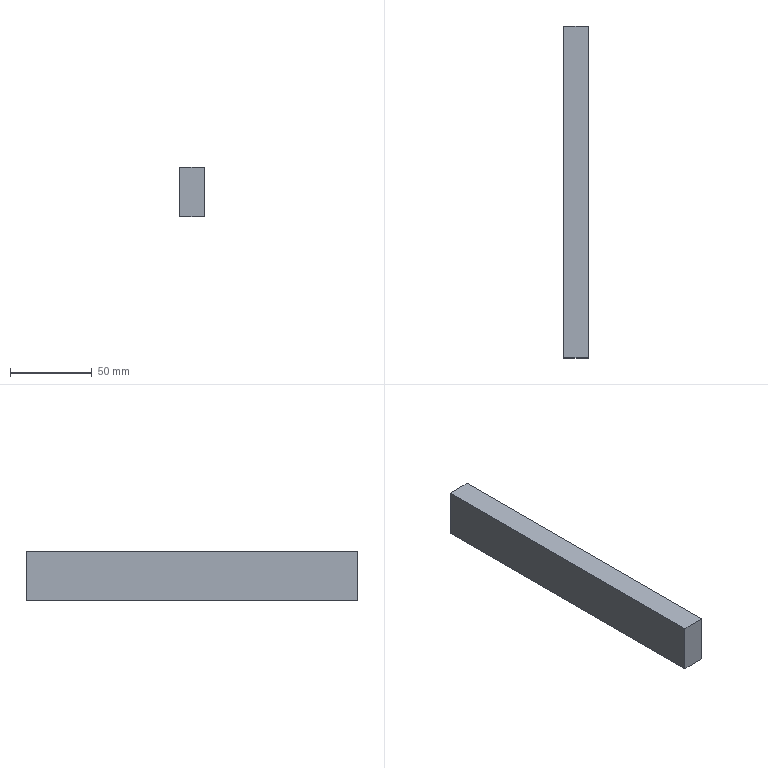Component | SolidWorks | SlideRailFixingPlate-1 | 1 solid | 6 faces | box 14.7 x 203 x 30 mm | volume 89523 mm3 | plane 6
build123d program:
from build123d import *

# Parameters (mm, degrees)
BOSS_EXTRUDE1_DEPTH      = 78
BOSS_EXTRUDE1_DEPTH_BACK = 125
SKETCH2_W                = 30
SKETCH2_H                = 14.7


with BuildPart() as part:
    # Sketch2 → Boss-Extrude1 (new, two sides: drawn at the far end of the back side and taken through both)
    with BuildSketch(Plane.XY.offset(-BOSS_EXTRUDE1_DEPTH_BACK)):
        with Locations((0, 243.349)):
            Rectangle(SKETCH2_W, SKETCH2_H)
    extrude(amount=BOSS_EXTRUDE1_DEPTH + BOSS_EXTRUDE1_DEPTH_BACK)


solid = part.part

# Placed as in the assembly
solid = solid.moved(Location((-235.297, 103.983, 271.626), (90, 0, 90)))
STEP:
#1=COLOUR_RGB('',0.7922,0.8196,0.9333);
#2=FILL_AREA_STYLE_COLOUR('',#1);
#3=FILL_AREA_STYLE('',(#2));
#4=SURFACE_STYLE_FILL_AREA(#3);
#5=SURFACE_SIDE_STYLE('',(#4));
#6=SURFACE_STYLE_USAGE(.BOTH.,#5);
#7=PRESENTATION_STYLE_ASSIGNMENT((#6));
#8=CARTESIAN_POINT('',(-19.134,1.023,11.284));
#9=VERTEX_POINT('',#8);
#10=CARTESIAN_POINT('',(-19.134,9.015,11.284));
#11=VERTEX_POINT('',#10);
#12=CARTESIAN_POINT('',(-19.134,1.023,11.284));
#13=DIRECTION('',(-0.,1.,-0.));
#14=VECTOR('',#13,39.37);
#15=LINE('',#12,#14);
#16=EDGE_CURVE('',#9,#11,#15,.T.);
#17=ORIENTED_EDGE('',*,*,#16,.T.);
#18=CARTESIAN_POINT('',(-19.134,9.015,10.103));
#19=VERTEX_POINT('',#18);
#20=CARTESIAN_POINT('',(-19.134,9.015,10.103));
#21=DIRECTION('',(-0.,0.,1.));
#22=VECTOR('',#21,39.37);
#23=LINE('',#20,#22);
#24=EDGE_CURVE('',#19,#11,#23,.T.);
#25=ORIENTED_EDGE('',*,*,#24,.F.);
#26=CARTESIAN_POINT('',(-19.134,1.023,10.103));
#27=VERTEX_POINT('',#26);
#28=CARTESIAN_POINT('',(-19.134,1.023,10.103));
#29=DIRECTION('',(-0.,1.,-0.));
#30=VECTOR('',#29,39.37);
#31=LINE('',#28,#30);
#32=EDGE_CURVE('',#27,#19,#31,.T.);
#33=ORIENTED_EDGE('',*,*,#32,.F.);
#34=CARTESIAN_POINT('',(-19.134,1.023,10.103));
#35=DIRECTION('',(-0.,0.,1.));
#36=VECTOR('',#35,39.37);
#37=LINE('',#34,#36);
#38=EDGE_CURVE('',#27,#9,#37,.T.);
#39=ORIENTED_EDGE('',*,*,#38,.T.);
#40=EDGE_LOOP('',(#17,#25,#33,#39));
#41=FACE_OUTER_BOUND('',#40,.T.);
#42=CARTESIAN_POINT('',(-19.134,1.023,10.103));
#43=DIRECTION('',(-1.,-0.,-0.));
#44=DIRECTION('',(-0.,1.,-0.));
#45=AXIS2_PLACEMENT_3D('',#42,#43,#44);
#46=PLANE('',#45);
#47=ADVANCED_FACE('',(#41),#46,.T.);
#48=ORIENTED_EDGE('',*,*,#32,.T.);
#49=CARTESIAN_POINT('',(-18.555,9.015,10.103));
#50=VERTEX_POINT('',#49);
#51=CARTESIAN_POINT('',(-18.555,9.015,10.103));
#52=DIRECTION('',(-1.,-0.,-0.));
#53=VECTOR('',#52,39.37);
#54=LINE('',#51,#53);
#55=EDGE_CURVE('',#50,#19,#54,.T.);
#56=ORIENTED_EDGE('',*,*,#55,.F.);
#57=CARTESIAN_POINT('',(-18.555,1.023,10.103));
#58=VERTEX_POINT('',#57);
#59=CARTESIAN_POINT('',(-18.555,1.023,10.103));
#60=DIRECTION('',(-0.,1.,-0.));
#61=VECTOR('',#60,39.37);
#62=LINE('',#59,#61);
#63=EDGE_CURVE('',#58,#50,#62,.T.);
#64=ORIENTED_EDGE('',*,*,#63,.F.);
#65=CARTESIAN_POINT('',(-18.555,1.023,10.103));
#66=DIRECTION('',(-1.,-0.,-0.));
#67=VECTOR('',#66,39.37);
#68=LINE('',#65,#67);
#69=EDGE_CURVE('',#58,#27,#68,.T.);
#70=ORIENTED_EDGE('',*,*,#69,.T.);
#71=EDGE_LOOP('',(#48,#56,#64,#70));
#72=FACE_OUTER_BOUND('',#71,.T.);
#73=CARTESIAN_POINT('',(-18.555,1.023,10.103));
#74=DIRECTION('',(0.,-0.,-1.));
#75=DIRECTION('',(0.,-1.,0.));
#76=AXIS2_PLACEMENT_3D('',#73,#74,#75);
#77=PLANE('',#76);
#78=ADVANCED_FACE('',(#72),#77,.T.);
#79=ORIENTED_EDGE('',*,*,#63,.T.);
#80=CARTESIAN_POINT('',(-18.555,9.015,11.284));
#81=VERTEX_POINT('',#80);
#82=CARTESIAN_POINT('',(-18.555,9.015,10.103));
#83=DIRECTION('',(-0.,0.,1.));
#84=VECTOR('',#83,39.37);
#85=LINE('',#82,#84);
#86=EDGE_CURVE('',#50,#81,#85,.T.);
#87=ORIENTED_EDGE('',*,*,#86,.T.);
#88=CARTESIAN_POINT('',(-18.555,1.023,11.284));
#89=VERTEX_POINT('',#88);
#90=CARTESIAN_POINT('',(-18.555,1.023,11.284));
#91=DIRECTION('',(-0.,1.,-0.));
#92=VECTOR('',#91,39.37);
#93=LINE('',#90,#92);
#94=EDGE_CURVE('',#89,#81,#93,.T.);
#95=ORIENTED_EDGE('',*,*,#94,.F.);
#96=CARTESIAN_POINT('',(-18.555,1.023,10.103));
#97=DIRECTION('',(-0.,0.,1.));
#98=VECTOR('',#97,39.37);
#99=LINE('',#96,#98);
#100=EDGE_CURVE('',#58,#89,#99,.T.);
#101=ORIENTED_EDGE('',*,*,#100,.F.);
#102=EDGE_LOOP('',(#79,#87,#95,#101));
#103=FACE_OUTER_BOUND('',#102,.T.);
#104=CARTESIAN_POINT('',(-18.555,1.023,10.103));
#105=DIRECTION('',(-1.,-0.,-0.));
#106=DIRECTION('',(-0.,1.,-0.));
#107=AXIS2_PLACEMENT_3D('',#104,#105,#106);
#108=PLANE('',#107);
#109=ADVANCED_FACE('',(#103),#108,.F.);
#110=ORIENTED_EDGE('',*,*,#94,.T.);
#111=CARTESIAN_POINT('',(-18.555,9.015,11.284));
#112=DIRECTION('',(-1.,-0.,-0.));
#113=VECTOR('',#112,39.37);
#114=LINE('',#111,#113);
#115=EDGE_CURVE('',#81,#11,#114,.T.);
#116=ORIENTED_EDGE('',*,*,#115,.T.);
#117=ORIENTED_EDGE('',*,*,#16,.F.);
#118=CARTESIAN_POINT('',(-18.555,1.023,11.284));
#119=DIRECTION('',(-1.,-0.,-0.));
#120=VECTOR('',#119,39.37);
#121=LINE('',#118,#120);
#122=EDGE_CURVE('',#89,#9,#121,.T.);
#123=ORIENTED_EDGE('',*,*,#122,.F.);
#124=EDGE_LOOP('',(#110,#116,#117,#123));
#125=FACE_OUTER_BOUND('',#124,.T.);
#126=CARTESIAN_POINT('',(-18.555,1.023,11.284));
#127=DIRECTION('',(0.,-0.,-1.));
#128=DIRECTION('',(0.,-1.,0.));
#129=AXIS2_PLACEMENT_3D('',#126,#127,#128);
#130=PLANE('',#129);
#131=ADVANCED_FACE('',(#125),#130,.F.);
#132=ORIENTED_EDGE('',*,*,#38,.F.);
#133=ORIENTED_EDGE('',*,*,#69,.F.);
#134=ORIENTED_EDGE('',*,*,#100,.T.);
#135=ORIENTED_EDGE('',*,*,#122,.T.);
#136=EDGE_LOOP('',(#132,#133,#134,#135));
#137=FACE_OUTER_BOUND('',#136,.T.);
#138=CARTESIAN_POINT('',(-9.264,1.023,10.694));
#139=DIRECTION('',(0.,-1.,0.));
#140=DIRECTION('',(-0.,0.,1.));
#141=AXIS2_PLACEMENT_3D('',#138,#139,#140);
#142=PLANE('',#141);
#143=ADVANCED_FACE('',(#137),#142,.T.);
#144=ORIENTED_EDGE('',*,*,#24,.T.);
#145=ORIENTED_EDGE('',*,*,#115,.F.);
#146=ORIENTED_EDGE('',*,*,#86,.F.);
#147=ORIENTED_EDGE('',*,*,#55,.T.);
#148=EDGE_LOOP('',(#144,#145,#146,#147));
#149=FACE_OUTER_BOUND('',#148,.T.);
#150=CARTESIAN_POINT('',(-9.264,9.015,10.694));
#151=DIRECTION('',(0.,-1.,0.));
#152=DIRECTION('',(-0.,0.,1.));
#153=AXIS2_PLACEMENT_3D('',#150,#151,#152);
#154=PLANE('',#153);
#155=ADVANCED_FACE('',(#149),#154,.F.);
#156=CLOSED_SHELL('',(#47,#78,#109,#131,#143,#155));
#157=MANIFOLD_SOLID_BREP('',#156);
#158=STYLED_ITEM('',(#7),#157);
#159=PRESENTATION_LAYER_ASSIGNMENT('','',(#158));
#160=CARTESIAN_POINT('',(0.,0.,0.));
#161=DIRECTION('',(0.,0.,1.));
#162=DIRECTION('',(1.,0.,0.));
#163=AXIS2_PLACEMENT_3D('',#160,#161,#162);
#164=(LENGTH_UNIT()NAMED_UNIT(*)SI_UNIT($,.METRE.));
#165=LENGTH_MEASURE_WITH_UNIT(LENGTH_MEASURE(0.0254),#164);
#166=DIMENSIONAL_EXPONENTS(1.,0.,0.,0.,0.,0.,0.);
#167=(CONVERSION_BASED_UNIT('',#165)LENGTH_UNIT()NAMED_UNIT(#166));
#168=UNCERTAINTY_MEASURE_WITH_UNIT(LENGTH_MEASURE(0.00001),#167,'','');
#169=(NAMED_UNIT(*)PLANE_ANGLE_UNIT()SI_UNIT($,.RADIAN.));
#170=(NAMED_UNIT(*)SI_UNIT($,.STERADIAN.)SOLID_ANGLE_UNIT());
#171=(GEOMETRIC_REPRESENTATION_CONTEXT(3)GLOBAL_UNCERTAINTY_ASSIGNED_CONTEXT((#168))GLOBAL_UNIT_ASSIGNED_CONTEXT((#167,#169,#170))REPRESENTATION_CONTEXT('',''));
#172=ADVANCED_BREP_SHAPE_REPRESENTATION('',(#157,#163),#171);
#173=(LENGTH_UNIT()NAMED_UNIT(*)SI_UNIT($,.METRE.));
#174=LENGTH_MEASURE_WITH_UNIT(LENGTH_MEASURE(0.0254),#173);
#175=DIMENSIONAL_EXPONENTS(1.,0.,0.,0.,0.,0.,0.);
#176=(CONVERSION_BASED_UNIT('',#174)LENGTH_UNIT()NAMED_UNIT(#175));
#177=UNCERTAINTY_MEASURE_WITH_UNIT(LENGTH_MEASURE(0.00001),#176,'','');
#178=(NAMED_UNIT(*)PLANE_ANGLE_UNIT()SI_UNIT($,.RADIAN.));
#179=(NAMED_UNIT(*)SI_UNIT($,.STERADIAN.)SOLID_ANGLE_UNIT());
#180=(GEOMETRIC_REPRESENTATION_CONTEXT(3)GLOBAL_UNCERTAINTY_ASSIGNED_CONTEXT((#177))GLOBAL_UNIT_ASSIGNED_CONTEXT((#176,#178,#179))REPRESENTATION_CONTEXT('',''));
#181=MECHANICAL_DESIGN_GEOMETRIC_PRESENTATION_REPRESENTATION('',(#158),#180);